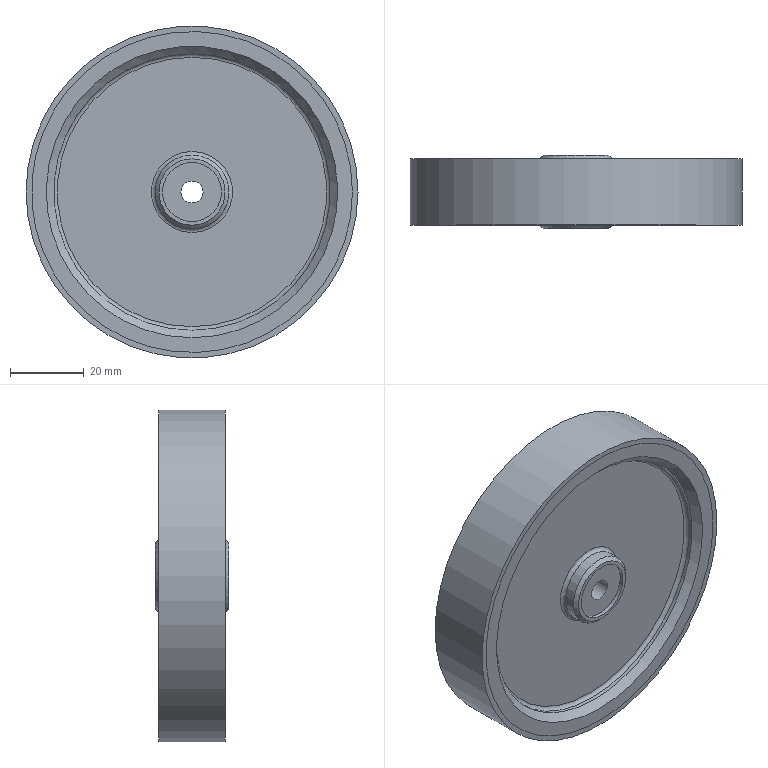Component | NX | UNI_WHEEL_BODY_2 | 2 solids | 28 faces | volume 80507 mm3 | cylinder 10 | plane 10 | cone 4 | torus 4 | commonest cylinder face diameters 87 x2 20 x2 16 x2 75 x2 90 x1 6 x1